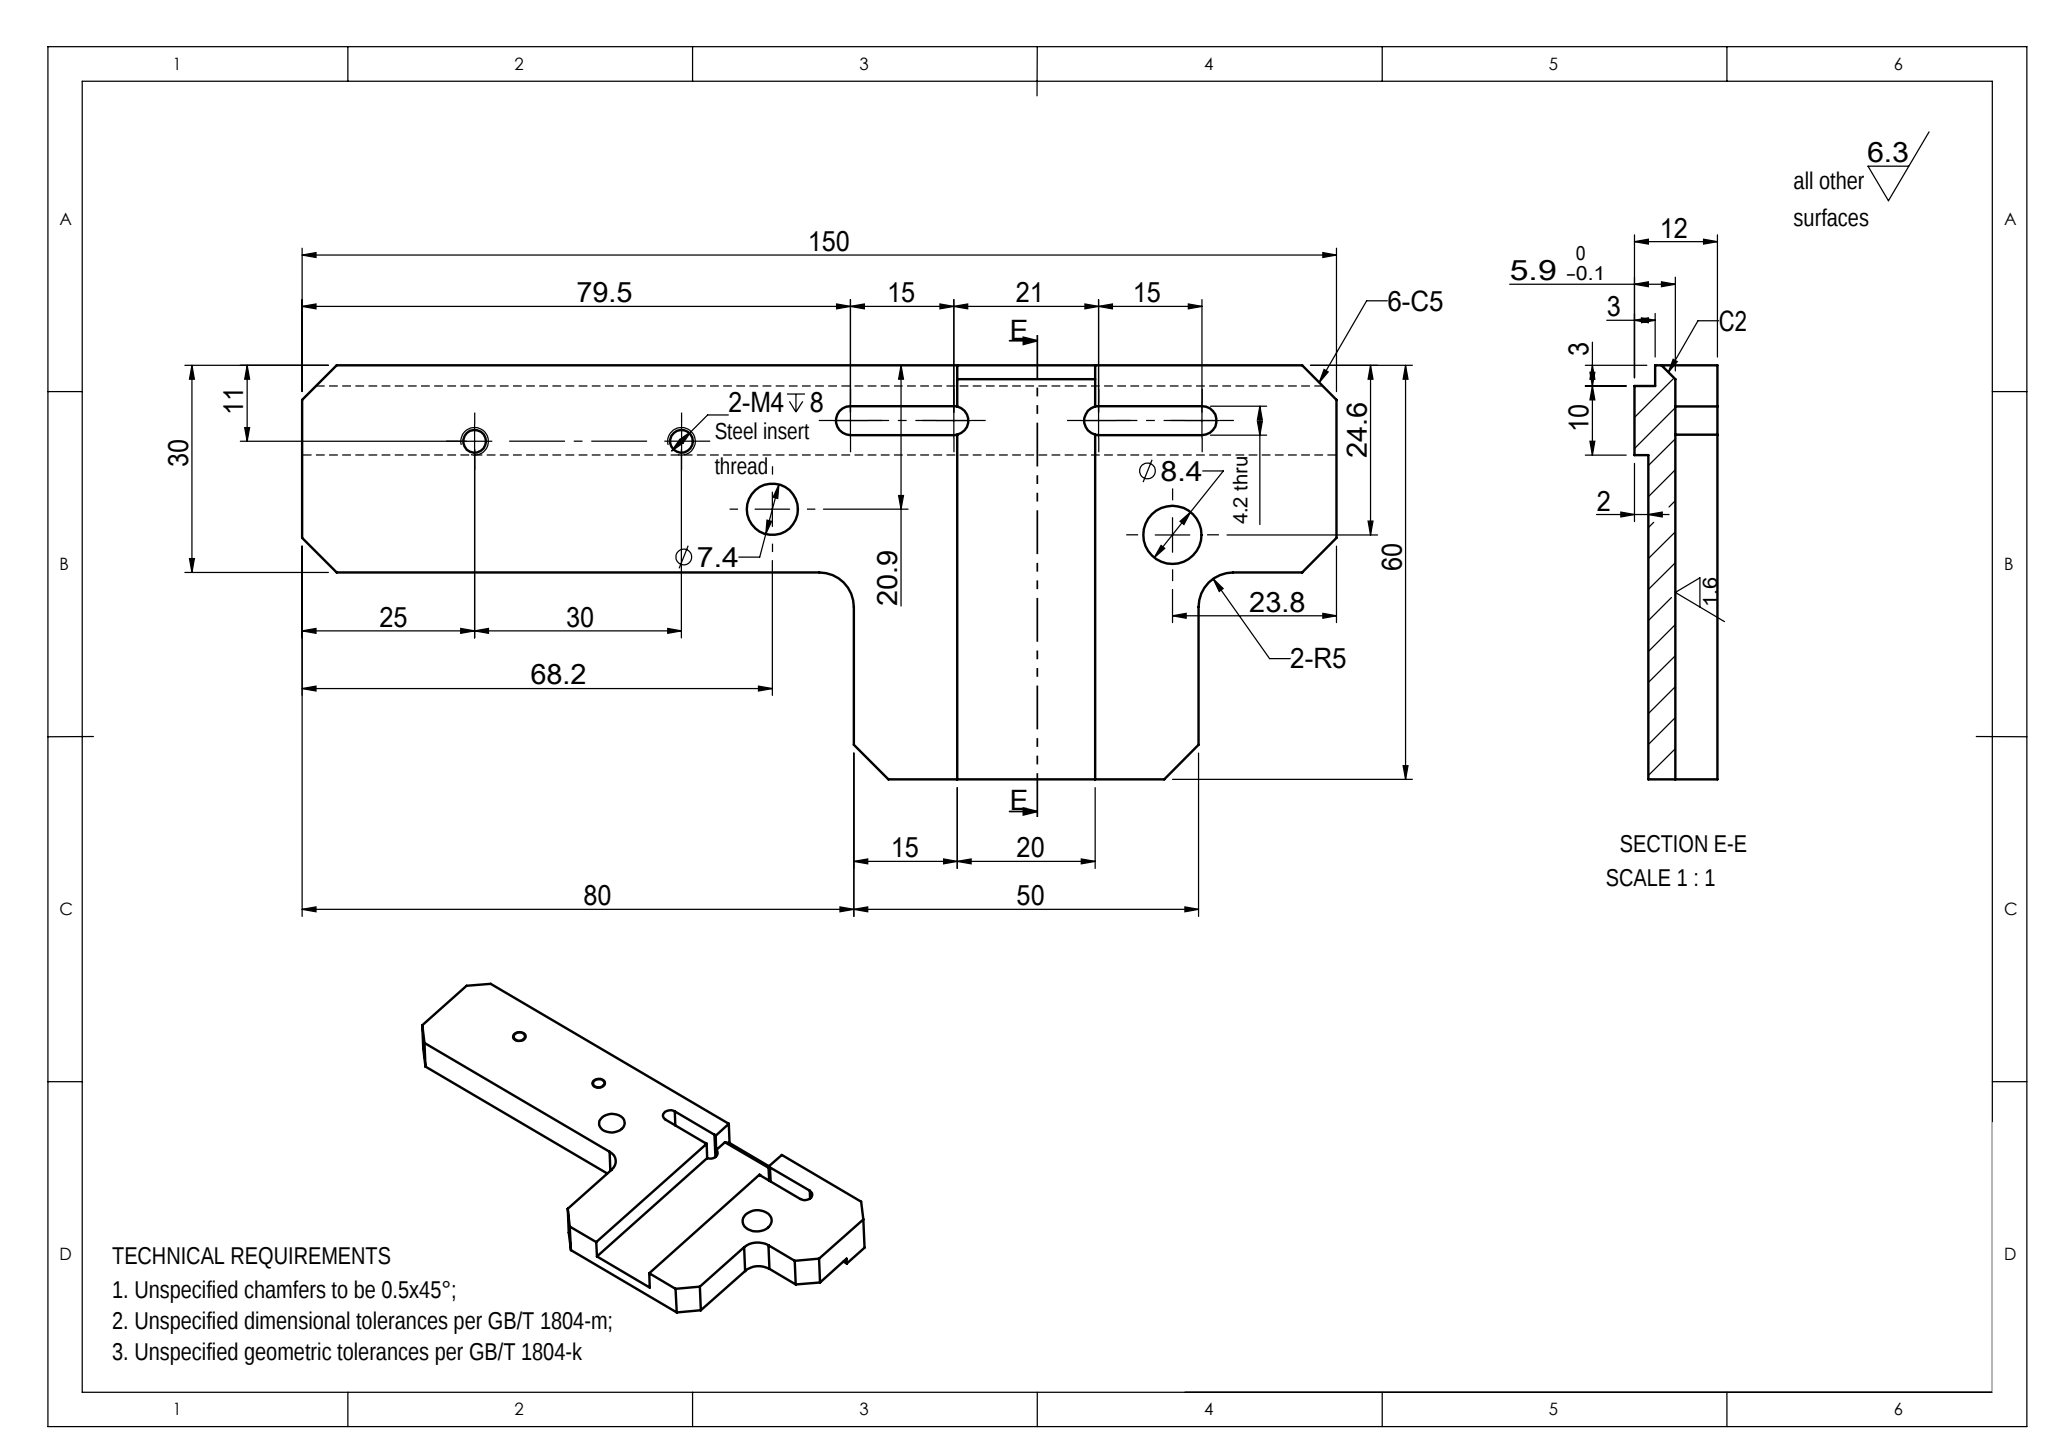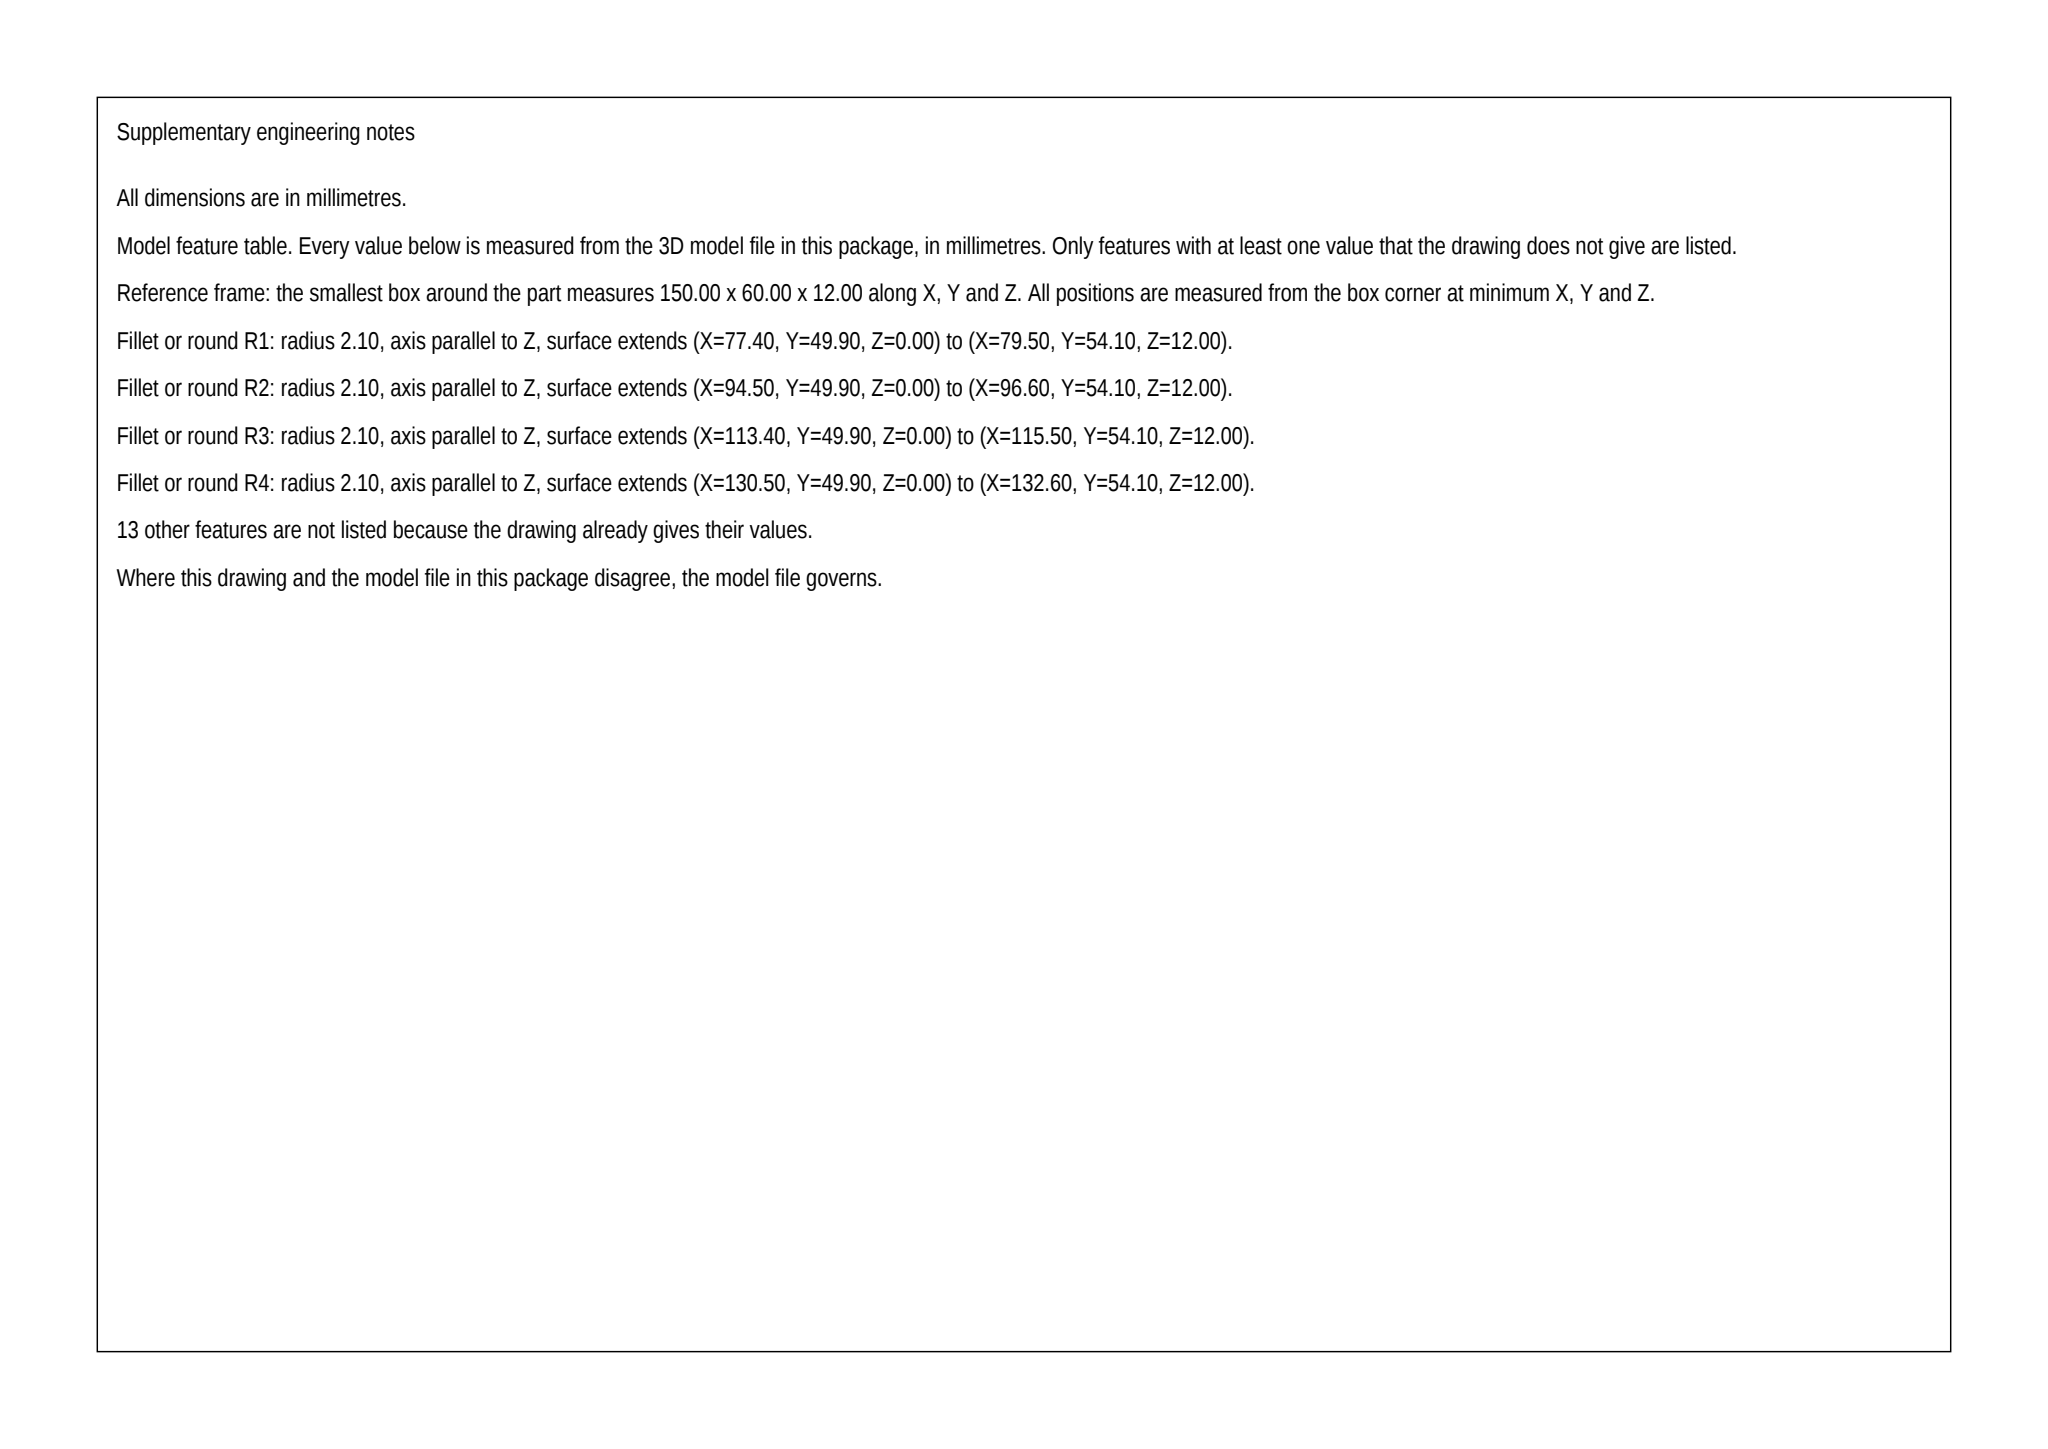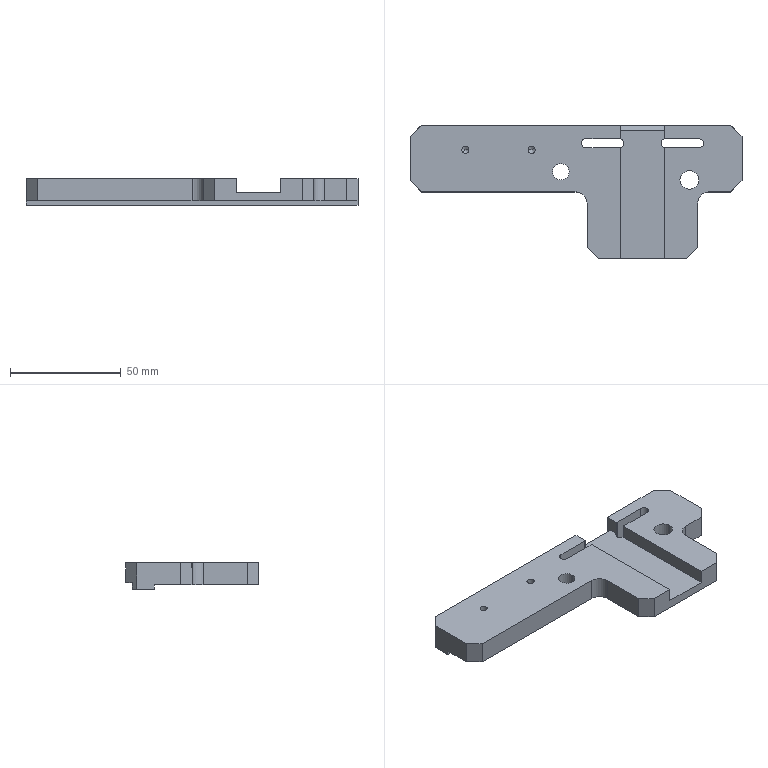Part | SolidWorks | mm | 1 solid | 51 faces | box 150 x 60 x 12 mm | volume 51603 mm3 | plane 31 | cylinder 16 | cone 4 | commonest cylinder face diameters 4.2 x6 3.3 x4 7.435 x2 8.438 x2 10 x2
build123d program:
from build123d import *

# Parameters (mm, degrees)
SKETCH1_W             = 150
SKETCH1_H             = 60
BOSS_EXTRUDE1_DEPTH   = 12
SKETCH2_W             = 3
SKETCH2_H             = 3
CUT_EXTRUDE1_DEPTH    = 154.441
CUT_EXTRUDE2_DEPTH    = 15.9
SKETCH10_W            = 2
SKETCH10_H            = 47
CUT_EXTRUDE7_DEPTH    = 154.441
SKETCH11_W            = 20
SKETCH11_H            = 83.59
CUT_EXTRUDE8_DEPTH    = 6.1
CHAMFER1_SIZE         = 2
SKETCH12_W            = 80
SKETCH12_H            = 30
SKETCH12_W_2          = 20
CUT_EXTRUDE9_DEPTH    = 45.9
CHAMFER2_SIZE         = 5
FILLET1_R             = 5
M4_TAPPED_HOLE1_D     = 3.3
M4_TAPPED_HOLE1_DEPTH = 10.1
M4_TAPPED_HOLE1_TIP   = 0.9914
SKETCH15_R            = 3.718
SKETCH15_R_2          = 4.219
CUT_EXTRUDE10_DEPTH   = 80


with BuildPart() as part:
    # Sketch1 → Boss-Extrude1 (new body)
    with BuildSketch(Plane.XY):
        Rectangle(SKETCH1_W, SKETCH1_H)
    extrude(amount=BOSS_EXTRUDE1_DEPTH)

    # Sketch2 → Cut-Extrude1 (cut, through all)
    with BuildSketch(Plane(origin=(75, 0, 0), x_dir=(0, 0, -1), z_dir=(1, 0, 0))):
        with Locations((-1.5, 28.5)):
            Rectangle(SKETCH2_W, SKETCH2_H)
    extrude(amount=-CUT_EXTRUDE1_DEPTH, mode=Mode.SUBTRACT)

    # Sketch3 → Cut-Extrude2 (cut)
    with BuildSketch(Plane.XY.offset(12)):
        with BuildLine():
            Line((4.5, 24.1), (19.5, 24.1))
            ThreePointArc((19.5, 24.1), (21.6, 22), (19.5, 19.9))
            Line((19.5, 19.9), (4.5, 19.9))
            ThreePointArc((4.5, 19.9), (2.4, 22), (4.5, 24.1))
        make_face()
        with BuildLine():
            Line((55.5, 24.1), (40.5, 24.1))
            ThreePointArc((40.5, 24.1), (38.4, 22), (40.5, 19.9))
            Line((40.5, 19.9), (55.5, 19.9))
            ThreePointArc((55.5, 19.9), (57.6, 22), (55.5, 24.1))
        make_face()
    extrude(amount=-CUT_EXTRUDE2_DEPTH, mode=Mode.SUBTRACT)

    # Sketch10 → Cut-Extrude7 (cut, through all)
    with BuildSketch(Plane.ZY.offset(75)):
        with Locations((1, -6.5)):
            Rectangle(SKETCH10_W, SKETCH10_H)
    extrude(amount=-CUT_EXTRUDE7_DEPTH, mode=Mode.SUBTRACT)

    # Sketch11 → Cut-Extrude8 (cut)
    with BuildSketch(Plane.XY.offset(12)):
        with Locations((30, 0.2846)):
            Rectangle(SKETCH11_W, SKETCH11_H)
    extrude(amount=-CUT_EXTRUDE8_DEPTH, mode=Mode.SUBTRACT)

    # Chamfer1
    chamfer1_edges = [part.edges().sort_by_distance(p)[0] for p in [
        (30, 30, 5.9),
    ]]
    chamfer(chamfer1_edges, length=CHAMFER1_SIZE)

    # Sketch12 → Cut-Extrude9 (cut)
    with BuildSketch(Plane.XY.offset(12)):
        with Locations((-35, -15)):
            Rectangle(SKETCH12_W, SKETCH12_H)
        with Locations((65, -15)):
            Rectangle(SKETCH12_W_2, SKETCH12_H)
    extrude(amount=-CUT_EXTRUDE9_DEPTH, mode=Mode.SUBTRACT)

    # Chamfer2
    chamfer2_edges = [part.edges().sort_by_distance(p)[0] for p in [
        (-75, 30, 7.5),
        (75, 30, 7.5),
        (-75, 0, 7),
        (75, 0, 7),
        (55, -30, 7),
        (5, -30, 7),
    ]]
    chamfer(chamfer2_edges, length=CHAMFER2_SIZE)

    # Fillet1
    fillet1_edges = [part.edges().sort_by_distance(p)[0] for p in [
        (5, 0, 7),
        (55, 0, 7),
    ]]
    fillet(fillet1_edges, radius=FILLET1_R)

    # M4 Tapped Hole1
    with Locations(Plane.XY.offset(12)):
        with Locations((-50, 19), (-20, 19)):
            Hole(M4_TAPPED_HOLE1_D / 2, depth=M4_TAPPED_HOLE1_DEPTH)
            with Locations((0, 0, -(M4_TAPPED_HOLE1_DEPTH + M4_TAPPED_HOLE1_TIP / 2))):  # 118° drill point
                Cone(0, M4_TAPPED_HOLE1_D / 2, M4_TAPPED_HOLE1_TIP, mode=Mode.SUBTRACT)

    # Sketch15 → Cut-Extrude10 (cut)
    with BuildSketch(Plane.XY.offset(12)):
        with Locations((-6.816, 9.15)):
            Circle(SKETCH15_R)
        with Locations((51.207, 5.432)):
            Circle(SKETCH15_R_2)
    extrude(amount=-CUT_EXTRUDE10_DEPTH, mode=Mode.SUBTRACT)


solid = part.part